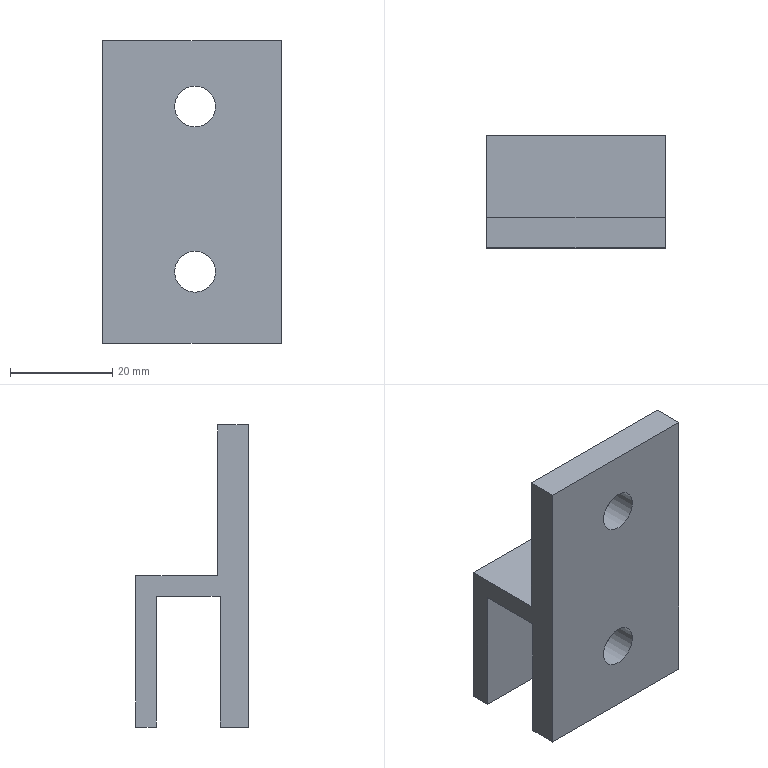Component | NX | CYL_MOUNT_PLATE | 1 solid | 16 faces | volume 16933 mm3 | plane 12 | cylinder 3 | cone 1 | commonest cylinder face diameters 8 x3